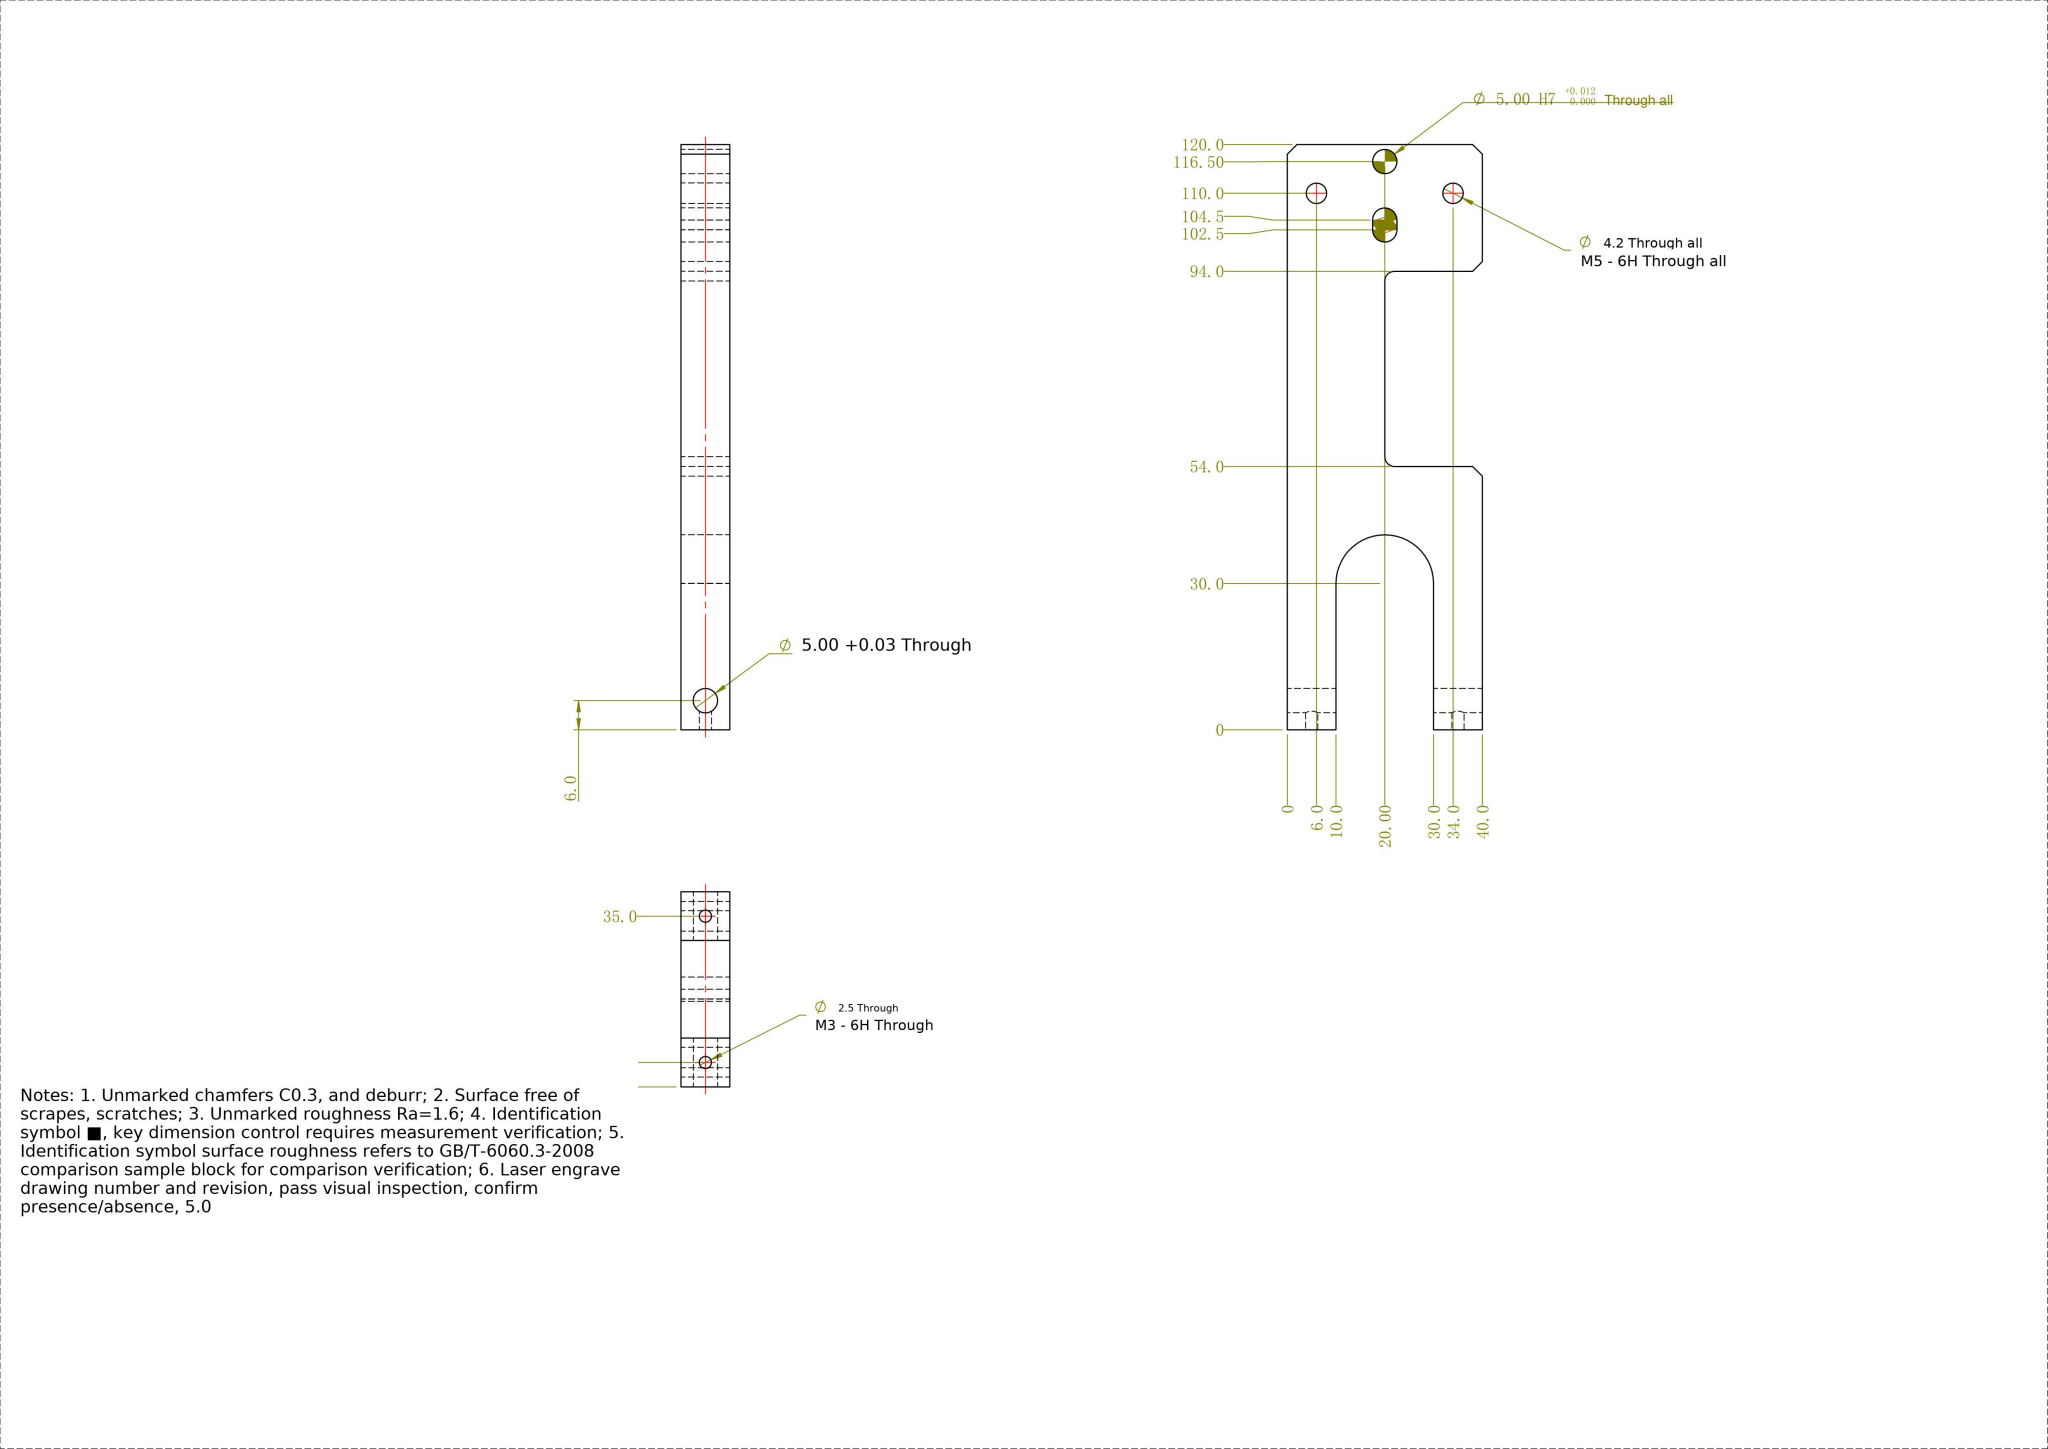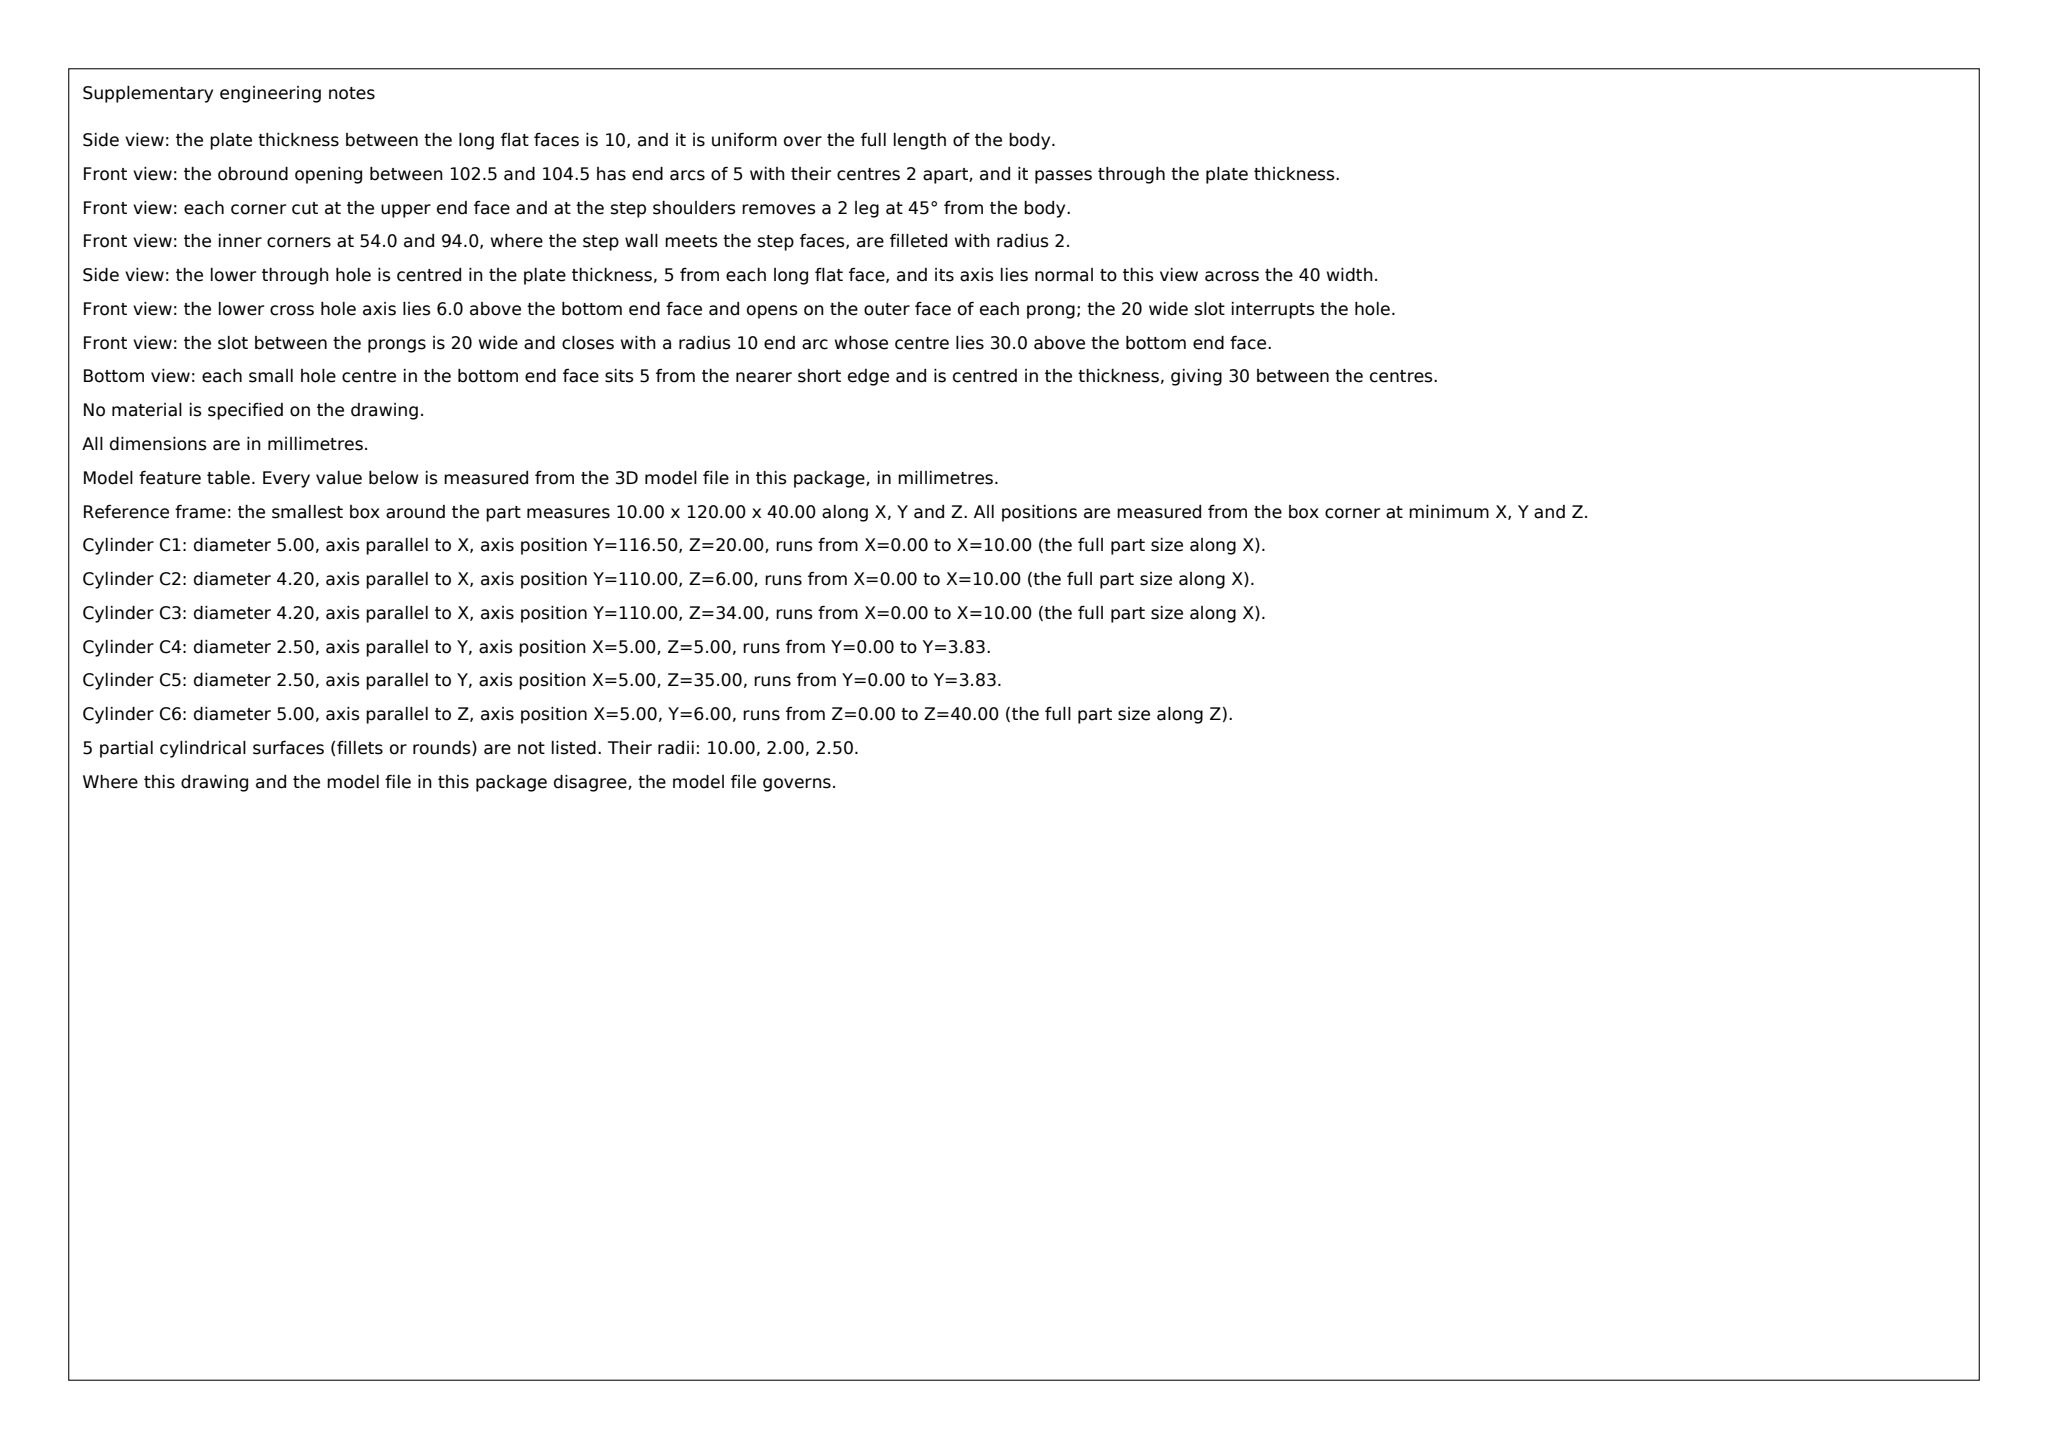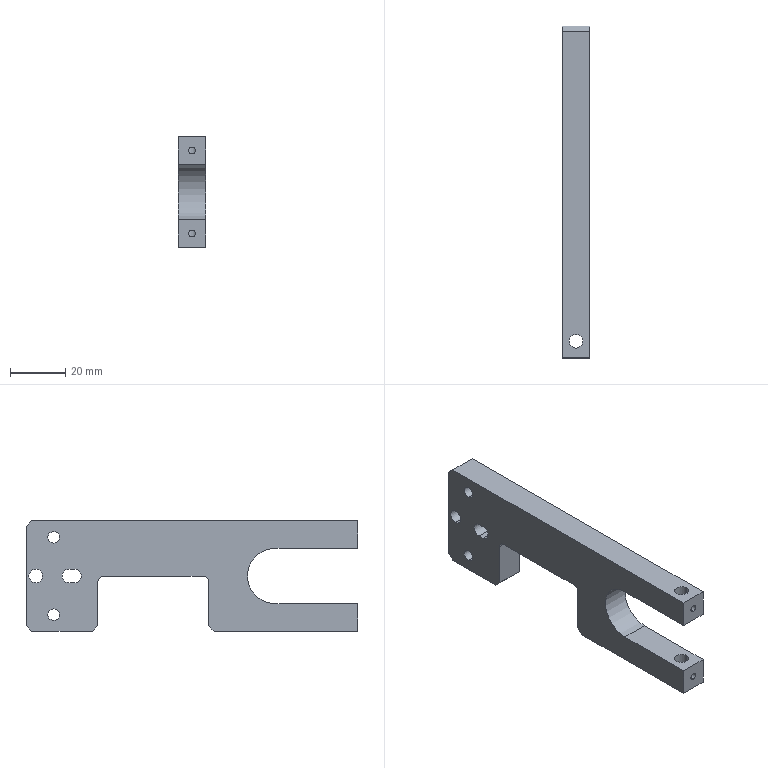Part | SolidWorks | mm | 1 solid | 39 faces | box 10 x 120 x 40 mm | volume 31169 mm3 | cylinder 20 | plane 19 | commonest cylinder face diameters 5 x9 4.2 x4 2.5 x4 4 x2 20 x1
Drawing notes:
Ø5.00 +0.03 & M3-6H HOLES ON CL: 5.0 FROM EA FACE, 10 THK | from the solid: Ø5 axis-Z cyl at x=5.0; Ø2.5 cyls at x=5.0; planes x=0 and x=10
LOWER M3-6H HOLE 5.0 FROM BOTTOM EDGE (0 DATUM); UPPER 35.0 | from the solid: Ø2.5 cyls axis Y at z=5.0 and z=35.0, L=3.84; bbox z=40
build123d program:
from build123d import *

# Parameters (mm, degrees)
SKETCH1_W                 = 10
SKETCH1_H                 = 120
BOSS_EXTRUDE1_DEPTH       = 20
CUT_EXTRUDE1_DEPTH        = 65.031
SKETCH3_R                 = 2.5
CUT_EXTRUDE2_DEPTH        = 73.284
M3_TAPPED_HOLE1_REACH     = 123.758
M3_TAPPED_HOLE1_BORE_R    = 1.25
M5_TAPPED_HOLE1_D         = 4.2
SIZE_MM_DOWEL_PIN_HOLE1_D = 5
CUT_EXTRUDE3_DEPTH        = 65.031
SKETCH11_W                = 20
SKETCH11_H                = 40
CUT_EXTRUDE4_DEPTH        = 65.031
CHAMFER1_SIZE             = 2
FILLET1_R                 = 2


with BuildPart() as part:
    # Sketch1 → Boss-Extrude1 (new, symmetric)
    with BuildSketch(Plane.XY):
        Rectangle(SKETCH1_W, SKETCH1_H)
    extrude(amount=BOSS_EXTRUDE1_DEPTH, both=True)

    # Sketch2 → Cut-Extrude1 (cut, through all)
    with BuildSketch(Plane.ZY.offset(5)):
        with BuildLine():
            Line((-10, -60), (-10, -30))
            ThreePointArc((-10, -30), (0, -20), (10, -30))
            Line((10, -30), (10, -60))
            ThreePointArc((10, -60), (0, -70), (-10, -60))
        make_face()
    extrude(amount=-CUT_EXTRUDE1_DEPTH, mode=Mode.SUBTRACT)

    # Sketch3 → Cut-Extrude2 (cut, through all)
    with BuildSketch(Plane(origin=(0, 0, -20), x_dir=(-1, 0, 0), z_dir=(0, 0, -1))):
        with Locations((0, -54)):
            Circle(SKETCH3_R)
    extrude(amount=-CUT_EXTRUDE2_DEPTH, mode=Mode.SUBTRACT)

    # M3 Tapped Hole1 bore → M3 Tapped Hole1 (cut, up to next)
    with BuildSketch(Plane(origin=(0, -60, 0), x_dir=(-1, 0, 0), z_dir=(0, -1, 0)), mode=Mode.PRIVATE) as m3_tapped_hole1_sk1:
        with Locations((0, -15)):
            Circle(M3_TAPPED_HOLE1_BORE_R)
    m3_tapped_hole1_tool1 = extrude(m3_tapped_hole1_sk1.sketch, amount=-M3_TAPPED_HOLE1_REACH, mode=Mode.PRIVATE) & part.part
    # M3 Tapped Hole1 bore → M3 Tapped Hole1 (cut, up to next)
    with BuildSketch(Plane(origin=(0, -60, 0), x_dir=(-1, 0, 0), z_dir=(0, -1, 0)), mode=Mode.PRIVATE) as m3_tapped_hole1_sk2:
        with Locations((0, 15)):
            Circle(M3_TAPPED_HOLE1_BORE_R)
    m3_tapped_hole1_tool2 = extrude(m3_tapped_hole1_sk2.sketch, amount=-M3_TAPPED_HOLE1_REACH, mode=Mode.PRIVATE) & part.part
    add(m3_tapped_hole1_tool1.solids().sort_by_distance((0, -60, 15))[0], mode=Mode.SUBTRACT)
    add(m3_tapped_hole1_tool2.solids().sort_by_distance((0, -60, -15))[0], mode=Mode.SUBTRACT)

    # M5 Tapped Hole1 (through all)
    with Locations(Plane.ZY.offset(5)):
        with Locations((14, 50), (-14, 50)):
            Hole(M5_TAPPED_HOLE1_D / 2)

    # Size mm Dowel Pin Hole1 (through all)
    with Locations(Plane.ZY.offset(5)):
        with Locations((0, 56.5), (0, 43.5)):
            Hole(SIZE_MM_DOWEL_PIN_HOLE1_D / 2)

    # Sketch10 → Cut-Extrude3 (cut, through all)
    with BuildSketch(Plane.ZY.offset(5)):
        with BuildLine():
            Line((-2.5, 42.5), (-2.5, 44.5))
            ThreePointArc((-2.5, 44.5), (0, 47), (2.5, 44.5))
            Line((2.5, 44.5), (2.5, 42.5))
            ThreePointArc((2.5, 42.5), (0, 40), (-2.5, 42.5))
        make_face()
    extrude(amount=-CUT_EXTRUDE3_DEPTH, mode=Mode.SUBTRACT)

    # Sketch11 → Cut-Extrude4 (cut, through all)
    with BuildSketch(Plane(origin=(5, 0, 0), x_dir=(0, 0, -1), z_dir=(1, 0, 0))):
        with Locations((10, 14)):
            Rectangle(SKETCH11_W, SKETCH11_H)
    extrude(amount=-CUT_EXTRUDE4_DEPTH, mode=Mode.SUBTRACT)

    # Chamfer1
    chamfer1_edges = [part.edges().sort_by_distance(p)[0] for p in [
        (0, 34, -20),
        (0, -6, -20),
        (0, 60, -20),
        (0, 60, 20),
    ]]
    chamfer(chamfer1_edges, length=CHAMFER1_SIZE)

    # Fillet1
    fillet1_edges = [part.edges().sort_by_distance(p)[0] for p in [
        (0, -6, 0),
        (0, 34, 0),
    ]]
    fillet(fillet1_edges, radius=FILLET1_R)


solid = part.part